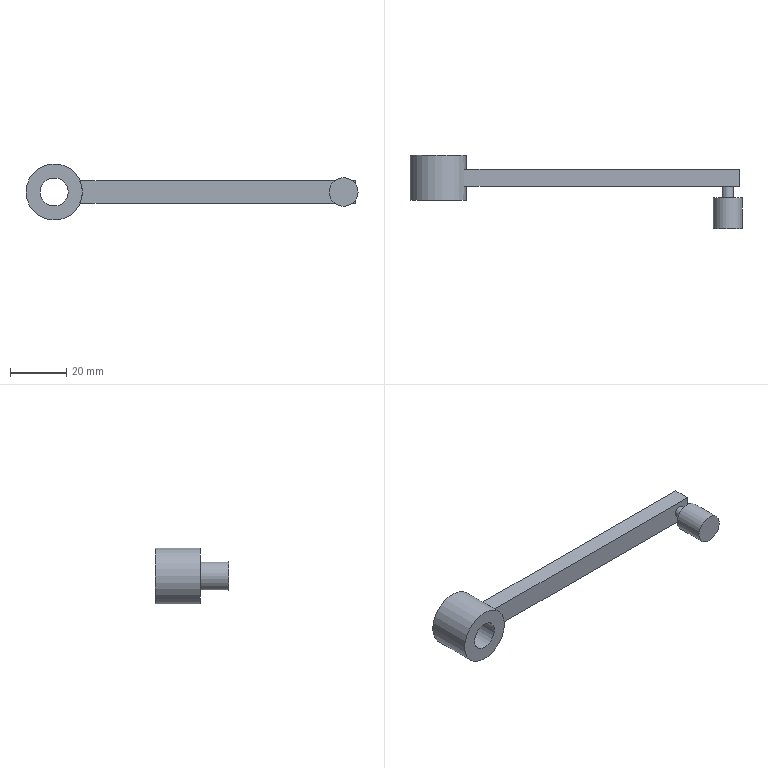Component | NX | HANDRAIL | 1 solid | 13 faces | box 117.89 x 26 x 20 mm | volume 9384 mm3 | plane 9 | cylinder 4 | commonest cylinder face diameters 20 x1 10 x1 4 x1 10.179 x1
STEP:
#1=CARTESIAN_POINT('',(0.,0.,0.));
#2=DIRECTION('',(0.,0.,1.));
#3=DIRECTION('',(1.,0.,0.));
#4=AXIS2_PLACEMENT_3D('',#1,#2,#3);
#5=CARTESIAN_POINT('',(-86.161,-205.381,46.));
#6=VERTEX_POINT('',#5);
#7=CARTESIAN_POINT('',(-86.161,-199.381,46.));
#8=VERTEX_POINT('',#7);
#9=CARTESIAN_POINT('',(-86.161,-210.381,46.));
#10=DIRECTION('',(0.,1.,0.));
#11=VECTOR('',#10,1.);
#12=LINE('',#9,#11);
#13=CARTESIAN_POINT('',(-95.326,-210.381,50.));
#14=DIRECTION('',(0.,1.,0.));
#15=DIRECTION('',(-1.,0.,0.));
#16=AXIS2_PLACEMENT_3D('',#13,#14,#15);
#17=CYLINDRICAL_SURFACE('',#16,10.);
#18=CARTESIAN_POINT('',(3.553,0.));
#19=DIRECTION('',(0.,1.));
#20=VECTOR('',#19,1.);
#21=LINE('',#18,#20);
#22=(GEOMETRIC_REPRESENTATION_CONTEXT(2)PARAMETRIC_REPRESENTATION_CONTEXT()REPRESENTATION_CONTEXT('',''));
#23=DEFINITIONAL_REPRESENTATION('',(#21),#22);
#24=PCURVE('',#17,#23);
#25=CARTESIAN_POINT('',(-88.326,-205.381,46.));
#26=DIRECTION('',(0.,0.,1.));
#27=DIRECTION('',(0.,-1.,0.));
#28=AXIS2_PLACEMENT_3D('',#25,#26,#27);
#29=PLANE('',#28);
#30=CARTESIAN_POINT('',(5.,2.165));
#31=DIRECTION('',(-1.,0.));
#32=VECTOR('',#31,1.);
#33=LINE('',#30,#32);
#34=(GEOMETRIC_REPRESENTATION_CONTEXT(2)PARAMETRIC_REPRESENTATION_CONTEXT()REPRESENTATION_CONTEXT('',''));
#35=DEFINITIONAL_REPRESENTATION('',(#33),#34);
#36=PCURVE('',#29,#35);
#37=SURFACE_CURVE('',#12,(#24,#36),.PCURVE_S1.);
#38=EDGE_CURVE('',#6,#8,#37,.T.);
#39=ORIENTED_EDGE('',*,*,#38,.F.);
#40=CARTESIAN_POINT('',(-85.326,-205.381,50.));
#41=VERTEX_POINT('',#40);
#42=CARTESIAN_POINT('',(-95.326,-205.381,50.));
#43=DIRECTION('',(0.,-1.,0.));
#44=DIRECTION('',(1.,0.,0.));
#45=AXIS2_PLACEMENT_3D('',#42,#43,#44);
#46=CIRCLE('',#45,10.);
#47=CARTESIAN_POINT('',(9.425,5.));
#48=DIRECTION('',(-1.,0.));
#49=VECTOR('',#48,1.);
#50=LINE('',#47,#49);
#51=(GEOMETRIC_REPRESENTATION_CONTEXT(2)PARAMETRIC_REPRESENTATION_CONTEXT()REPRESENTATION_CONTEXT('',''));
#52=DEFINITIONAL_REPRESENTATION('',(#50),#51);
#53=PCURVE('',#17,#52);
#54=CARTESIAN_POINT('',(-95.326,-205.381,50.));
#55=DIRECTION('',(0.,-1.,0.));
#56=DIRECTION('',(1.,0.,0.));
#57=AXIS2_PLACEMENT_3D('',#54,#55,#56);
#58=PLANE('',#57);
#59=CARTESIAN_POINT('',(0.,0.));
#60=DIRECTION('',(1.,0.));
#61=AXIS2_PLACEMENT_2D('',#59,#60);
#62=CIRCLE('',#61,10.);
#63=(GEOMETRIC_REPRESENTATION_CONTEXT(2)PARAMETRIC_REPRESENTATION_CONTEXT()REPRESENTATION_CONTEXT('',''));
#64=DEFINITIONAL_REPRESENTATION('',(#62),#63);
#65=PCURVE('',#58,#64);
#66=SURFACE_CURVE('',#46,(#53,#65),.PCURVE_S1.);
#67=EDGE_CURVE('',#6,#41,#66,.T.);
#68=ORIENTED_EDGE('',*,*,#67,.T.);
#69=CARTESIAN_POINT('',(-85.326,-210.381,50.));
#70=VERTEX_POINT('',#69);
#71=CARTESIAN_POINT('',(-85.326,-210.381,50.));
#72=CARTESIAN_POINT('',(-85.326,-205.381,50.));
#73=B_SPLINE_CURVE_WITH_KNOTS('',1,(#71,#72),.UNSPECIFIED.,.F.,.F.,(2,2),(0.,5.),.PIECEWISE_BEZIER_KNOTS.);
#74=CARTESIAN_POINT('',(3.142,0.));
#75=DIRECTION('',(0.,1.));
#76=VECTOR('',#75,1.);
#77=LINE('',#74,#76);
#78=(GEOMETRIC_REPRESENTATION_CONTEXT(2)PARAMETRIC_REPRESENTATION_CONTEXT()REPRESENTATION_CONTEXT('',''));
#79=DEFINITIONAL_REPRESENTATION('',(#77),#78);
#80=PCURVE('',#17,#79);
#81=CARTESIAN_POINT('',(9.425,0.));
#82=DIRECTION('',(0.,1.));
#83=VECTOR('',#82,1.);
#84=LINE('',#81,#83);
#85=(GEOMETRIC_REPRESENTATION_CONTEXT(2)PARAMETRIC_REPRESENTATION_CONTEXT()REPRESENTATION_CONTEXT('',''));
#86=DEFINITIONAL_REPRESENTATION('',(#84),#85);
#87=PCURVE('',#17,#86);
#88=SEAM_CURVE('',#73,(#80,#87),.PCURVE_S1.);
#89=EDGE_CURVE('',#70,#41,#88,.T.);
#90=ORIENTED_EDGE('',*,*,#89,.F.);
#91=CARTESIAN_POINT('',(-95.326,-210.381,50.));
#92=DIRECTION('',(0.,-1.,0.));
#93=DIRECTION('',(1.,0.,0.));
#94=AXIS2_PLACEMENT_3D('',#91,#92,#93);
#95=CIRCLE('',#94,10.);
#96=CARTESIAN_POINT('',(9.425,0.));
#97=DIRECTION('',(-1.,0.));
#98=VECTOR('',#97,1.);
#99=LINE('',#96,#98);
#100=(GEOMETRIC_REPRESENTATION_CONTEXT(2)PARAMETRIC_REPRESENTATION_CONTEXT()REPRESENTATION_CONTEXT('',''));
#101=DEFINITIONAL_REPRESENTATION('',(#99),#100);
#102=PCURVE('',#17,#101);
#103=CARTESIAN_POINT('',(-95.326,-210.381,50.));
#104=DIRECTION('',(0.,-1.,0.));
#105=DIRECTION('',(1.,0.,0.));
#106=AXIS2_PLACEMENT_3D('',#103,#104,#105);
#107=PLANE('',#106);
#108=CARTESIAN_POINT('',(0.,0.));
#109=DIRECTION('',(1.,0.));
#110=AXIS2_PLACEMENT_2D('',#108,#109);
#111=CIRCLE('',#110,10.);
#112=(GEOMETRIC_REPRESENTATION_CONTEXT(2)PARAMETRIC_REPRESENTATION_CONTEXT()REPRESENTATION_CONTEXT('',''));
#113=DEFINITIONAL_REPRESENTATION('',(#111),#112);
#114=PCURVE('',#107,#113);
#115=SURFACE_CURVE('',#95,(#102,#114),.PCURVE_S1.);
#116=EDGE_CURVE('',#70,#70,#115,.T.);
#117=ORIENTED_EDGE('',*,*,#116,.F.);
#118=ORIENTED_EDGE('',*,*,#89,.T.);
#119=CARTESIAN_POINT('',(-86.161,-205.381,54.));
#120=VERTEX_POINT('',#119);
#121=CARTESIAN_POINT('',(-95.326,-205.381,50.));
#122=DIRECTION('',(0.,-1.,0.));
#123=DIRECTION('',(1.,0.,0.));
#124=AXIS2_PLACEMENT_3D('',#121,#122,#123);
#125=CIRCLE('',#124,10.);
#126=CARTESIAN_POINT('',(15.708,5.));
#127=DIRECTION('',(-1.,0.));
#128=VECTOR('',#127,1.);
#129=LINE('',#126,#128);
#130=(GEOMETRIC_REPRESENTATION_CONTEXT(2)PARAMETRIC_REPRESENTATION_CONTEXT()REPRESENTATION_CONTEXT('',''));
#131=DEFINITIONAL_REPRESENTATION('',(#129),#130);
#132=PCURVE('',#17,#131);
#133=CARTESIAN_POINT('',(0.,0.));
#134=DIRECTION('',(1.,0.));
#135=AXIS2_PLACEMENT_2D('',#133,#134);
#136=CIRCLE('',#135,10.);
#137=(GEOMETRIC_REPRESENTATION_CONTEXT(2)PARAMETRIC_REPRESENTATION_CONTEXT()REPRESENTATION_CONTEXT('',''));
#138=DEFINITIONAL_REPRESENTATION('',(#136),#137);
#139=PCURVE('',#58,#138);
#140=SURFACE_CURVE('',#125,(#132,#139),.PCURVE_S1.);
#141=EDGE_CURVE('',#41,#120,#140,.T.);
#142=ORIENTED_EDGE('',*,*,#141,.T.);
#143=CARTESIAN_POINT('',(-86.161,-199.381,54.));
#144=VERTEX_POINT('',#143);
#145=CARTESIAN_POINT('',(-86.161,-210.381,54.));
#146=DIRECTION('',(0.,-1.,0.));
#147=VECTOR('',#146,1.);
#148=LINE('',#145,#147);
#149=CARTESIAN_POINT('',(9.013,0.));
#150=DIRECTION('',(0.,-1.));
#151=VECTOR('',#150,1.);
#152=LINE('',#149,#151);
#153=(GEOMETRIC_REPRESENTATION_CONTEXT(2)PARAMETRIC_REPRESENTATION_CONTEXT()REPRESENTATION_CONTEXT('',''));
#154=DEFINITIONAL_REPRESENTATION('',(#152),#153);
#155=PCURVE('',#17,#154);
#156=CARTESIAN_POINT('',(11.674,-205.381,54.));
#157=DIRECTION('',(0.,0.,-1.));
#158=DIRECTION('',(0.,1.,0.));
#159=AXIS2_PLACEMENT_3D('',#156,#157,#158);
#160=PLANE('',#159);
#161=CARTESIAN_POINT('',(-5.,-97.835));
#162=DIRECTION('',(-1.,0.));
#163=VECTOR('',#162,1.);
#164=LINE('',#161,#163);
#165=(GEOMETRIC_REPRESENTATION_CONTEXT(2)PARAMETRIC_REPRESENTATION_CONTEXT()REPRESENTATION_CONTEXT('',''));
#166=DEFINITIONAL_REPRESENTATION('',(#164),#165);
#167=PCURVE('',#160,#166);
#168=SURFACE_CURVE('',#148,(#155,#167),.PCURVE_S1.);
#169=EDGE_CURVE('',#144,#120,#168,.T.);
#170=ORIENTED_EDGE('',*,*,#169,.F.);
#171=CARTESIAN_POINT('',(-85.326,-199.381,50.));
#172=VERTEX_POINT('',#171);
#173=CARTESIAN_POINT('',(-95.326,-199.381,50.));
#174=DIRECTION('',(0.,-1.,0.));
#175=DIRECTION('',(1.,0.,0.));
#176=AXIS2_PLACEMENT_3D('',#173,#174,#175);
#177=CIRCLE('',#176,10.);
#178=CARTESIAN_POINT('',(15.708,11.));
#179=DIRECTION('',(-1.,0.));
#180=VECTOR('',#179,1.);
#181=LINE('',#178,#180);
#182=(GEOMETRIC_REPRESENTATION_CONTEXT(2)PARAMETRIC_REPRESENTATION_CONTEXT()REPRESENTATION_CONTEXT('',''));
#183=DEFINITIONAL_REPRESENTATION('',(#181),#182);
#184=PCURVE('',#17,#183);
#185=CARTESIAN_POINT('',(-95.326,-199.381,50.));
#186=DIRECTION('',(0.,-1.,0.));
#187=DIRECTION('',(1.,0.,0.));
#188=AXIS2_PLACEMENT_3D('',#185,#186,#187);
#189=PLANE('',#188);
#190=CARTESIAN_POINT('',(0.,0.));
#191=DIRECTION('',(1.,0.));
#192=AXIS2_PLACEMENT_2D('',#190,#191);
#193=CIRCLE('',#192,10.);
#194=(GEOMETRIC_REPRESENTATION_CONTEXT(2)PARAMETRIC_REPRESENTATION_CONTEXT()REPRESENTATION_CONTEXT('',''));
#195=DEFINITIONAL_REPRESENTATION('',(#193),#194);
#196=PCURVE('',#189,#195);
#197=SURFACE_CURVE('',#177,(#184,#196),.PCURVE_S1.);
#198=EDGE_CURVE('',#172,#144,#197,.T.);
#199=ORIENTED_EDGE('',*,*,#198,.F.);
#200=CARTESIAN_POINT('',(-85.326,-194.381,50.));
#201=VERTEX_POINT('',#200);
#202=CARTESIAN_POINT('',(-85.326,-199.381,50.));
#203=CARTESIAN_POINT('',(-85.326,-194.381,50.));
#204=B_SPLINE_CURVE_WITH_KNOTS('',1,(#202,#203),.UNSPECIFIED.,.F.,.F.,(2,2),(11.,16.),.PIECEWISE_BEZIER_KNOTS.);
#205=CARTESIAN_POINT('',(9.425,0.));
#206=DIRECTION('',(0.,1.));
#207=VECTOR('',#206,1.);
#208=LINE('',#205,#207);
#209=(GEOMETRIC_REPRESENTATION_CONTEXT(2)PARAMETRIC_REPRESENTATION_CONTEXT()REPRESENTATION_CONTEXT('',''));
#210=DEFINITIONAL_REPRESENTATION('',(#208),#209);
#211=PCURVE('',#17,#210);
#212=CARTESIAN_POINT('',(3.142,0.));
#213=DIRECTION('',(0.,1.));
#214=VECTOR('',#213,1.);
#215=LINE('',#212,#214);
#216=(GEOMETRIC_REPRESENTATION_CONTEXT(2)PARAMETRIC_REPRESENTATION_CONTEXT()REPRESENTATION_CONTEXT('',''));
#217=DEFINITIONAL_REPRESENTATION('',(#215),#216);
#218=PCURVE('',#17,#217);
#219=SEAM_CURVE('',#204,(#211,#218),.PCURVE_S1.);
#220=EDGE_CURVE('',#172,#201,#219,.T.);
#221=ORIENTED_EDGE('',*,*,#220,.T.);
#222=CARTESIAN_POINT('',(-95.326,-194.381,50.));
#223=DIRECTION('',(0.,-1.,0.));
#224=DIRECTION('',(1.,0.,0.));
#225=AXIS2_PLACEMENT_3D('',#222,#223,#224);
#226=CIRCLE('',#225,10.);
#227=CARTESIAN_POINT('',(9.425,16.));
#228=DIRECTION('',(-1.,0.));
#229=VECTOR('',#228,1.);
#230=LINE('',#227,#229);
#231=(GEOMETRIC_REPRESENTATION_CONTEXT(2)PARAMETRIC_REPRESENTATION_CONTEXT()REPRESENTATION_CONTEXT('',''));
#232=DEFINITIONAL_REPRESENTATION('',(#230),#231);
#233=PCURVE('',#17,#232);
#234=CARTESIAN_POINT('',(-95.326,-194.381,50.));
#235=DIRECTION('',(0.,-1.,0.));
#236=DIRECTION('',(1.,0.,0.));
#237=AXIS2_PLACEMENT_3D('',#234,#235,#236);
#238=PLANE('',#237);
#239=CARTESIAN_POINT('',(0.,0.));
#240=DIRECTION('',(1.,0.));
#241=AXIS2_PLACEMENT_2D('',#239,#240);
#242=CIRCLE('',#241,10.);
#243=(GEOMETRIC_REPRESENTATION_CONTEXT(2)PARAMETRIC_REPRESENTATION_CONTEXT()REPRESENTATION_CONTEXT('',''));
#244=DEFINITIONAL_REPRESENTATION('',(#242),#243);
#245=PCURVE('',#238,#244);
#246=SURFACE_CURVE('',#226,(#233,#245),.PCURVE_S1.);
#247=EDGE_CURVE('',#201,#201,#246,.T.);
#248=ORIENTED_EDGE('',*,*,#247,.T.);
#249=ORIENTED_EDGE('',*,*,#220,.F.);
#250=CARTESIAN_POINT('',(-95.326,-199.381,50.));
#251=DIRECTION('',(0.,-1.,0.));
#252=DIRECTION('',(1.,0.,0.));
#253=AXIS2_PLACEMENT_3D('',#250,#251,#252);
#254=CIRCLE('',#253,10.);
#255=CARTESIAN_POINT('',(9.425,11.));
#256=DIRECTION('',(-1.,0.));
#257=VECTOR('',#256,1.);
#258=LINE('',#255,#257);
#259=(GEOMETRIC_REPRESENTATION_CONTEXT(2)PARAMETRIC_REPRESENTATION_CONTEXT()REPRESENTATION_CONTEXT('',''));
#260=DEFINITIONAL_REPRESENTATION('',(#258),#259);
#261=PCURVE('',#17,#260);
#262=CARTESIAN_POINT('',(0.,0.));
#263=DIRECTION('',(1.,0.));
#264=AXIS2_PLACEMENT_2D('',#262,#263);
#265=CIRCLE('',#264,10.);
#266=(GEOMETRIC_REPRESENTATION_CONTEXT(2)PARAMETRIC_REPRESENTATION_CONTEXT()REPRESENTATION_CONTEXT('',''));
#267=DEFINITIONAL_REPRESENTATION('',(#265),#266);
#268=PCURVE('',#189,#267);
#269=SURFACE_CURVE('',#254,(#261,#268),.PCURVE_S1.);
#270=EDGE_CURVE('',#8,#172,#269,.T.);
#271=ORIENTED_EDGE('',*,*,#270,.F.);
#272=EDGE_LOOP('',(#39,#68,#90,#117,#118,#142,#170,#199,#221,#248,#249,#271));
#273=FACE_BOUND('',#272,.T.);
#274=ADVANCED_FACE('',(#273),#17,.T.);
#275=CARTESIAN_POINT('',(-90.326,-210.381,50.));
#276=VERTEX_POINT('',#275);
#277=CARTESIAN_POINT('',(-95.326,-210.381,50.));
#278=DIRECTION('',(0.,-1.,0.));
#279=DIRECTION('',(1.,0.,0.));
#280=AXIS2_PLACEMENT_3D('',#277,#278,#279);
#281=CIRCLE('',#280,5.);
#282=CARTESIAN_POINT('',(-95.326,-210.381,50.));
#283=DIRECTION('',(0.,1.,0.));
#284=DIRECTION('',(-1.,0.,0.));
#285=AXIS2_PLACEMENT_3D('',#282,#283,#284);
#286=CYLINDRICAL_SURFACE('',#285,5.);
#287=CARTESIAN_POINT('',(9.425,0.));
#288=DIRECTION('',(-1.,0.));
#289=VECTOR('',#288,1.);
#290=LINE('',#287,#289);
#291=(GEOMETRIC_REPRESENTATION_CONTEXT(2)PARAMETRIC_REPRESENTATION_CONTEXT()REPRESENTATION_CONTEXT('',''));
#292=DEFINITIONAL_REPRESENTATION('',(#290),#291);
#293=PCURVE('',#286,#292);
#294=CARTESIAN_POINT('',(0.,0.));
#295=DIRECTION('',(1.,0.));
#296=AXIS2_PLACEMENT_2D('',#294,#295);
#297=CIRCLE('',#296,5.);
#298=(GEOMETRIC_REPRESENTATION_CONTEXT(2)PARAMETRIC_REPRESENTATION_CONTEXT()REPRESENTATION_CONTEXT('',''));
#299=DEFINITIONAL_REPRESENTATION('',(#297),#298);
#300=PCURVE('',#107,#299);
#301=SURFACE_CURVE('',#281,(#293,#300),.PCURVE_S1.);
#302=EDGE_CURVE('',#276,#276,#301,.T.);
#303=ORIENTED_EDGE('',*,*,#302,.F.);
#304=CARTESIAN_POINT('',(-90.326,-194.381,50.));
#305=VERTEX_POINT('',#304);
#306=CARTESIAN_POINT('',(-90.326,-210.381,50.));
#307=CARTESIAN_POINT('',(-90.326,-194.381,50.));
#308=B_SPLINE_CURVE_WITH_KNOTS('',1,(#306,#307),.UNSPECIFIED.,.F.,.F.,(2,2),(0.,16.),.PIECEWISE_BEZIER_KNOTS.);
#309=CARTESIAN_POINT('',(9.425,0.));
#310=DIRECTION('',(0.,1.));
#311=VECTOR('',#310,1.);
#312=LINE('',#309,#311);
#313=(GEOMETRIC_REPRESENTATION_CONTEXT(2)PARAMETRIC_REPRESENTATION_CONTEXT()REPRESENTATION_CONTEXT('',''));
#314=DEFINITIONAL_REPRESENTATION('',(#312),#313);
#315=PCURVE('',#286,#314);
#316=CARTESIAN_POINT('',(3.142,0.));
#317=DIRECTION('',(0.,1.));
#318=VECTOR('',#317,1.);
#319=LINE('',#316,#318);
#320=(GEOMETRIC_REPRESENTATION_CONTEXT(2)PARAMETRIC_REPRESENTATION_CONTEXT()REPRESENTATION_CONTEXT('',''));
#321=DEFINITIONAL_REPRESENTATION('',(#319),#320);
#322=PCURVE('',#286,#321);
#323=SEAM_CURVE('',#308,(#315,#322),.PCURVE_S1.);
#324=EDGE_CURVE('',#276,#305,#323,.T.);
#325=ORIENTED_EDGE('',*,*,#324,.T.);
#326=CARTESIAN_POINT('',(-95.326,-194.381,50.));
#327=DIRECTION('',(0.,-1.,0.));
#328=DIRECTION('',(1.,0.,0.));
#329=AXIS2_PLACEMENT_3D('',#326,#327,#328);
#330=CIRCLE('',#329,5.);
#331=CARTESIAN_POINT('',(9.425,16.));
#332=DIRECTION('',(-1.,0.));
#333=VECTOR('',#332,1.);
#334=LINE('',#331,#333);
#335=(GEOMETRIC_REPRESENTATION_CONTEXT(2)PARAMETRIC_REPRESENTATION_CONTEXT()REPRESENTATION_CONTEXT('',''));
#336=DEFINITIONAL_REPRESENTATION('',(#334),#335);
#337=PCURVE('',#286,#336);
#338=CARTESIAN_POINT('',(0.,0.));
#339=DIRECTION('',(1.,0.));
#340=AXIS2_PLACEMENT_2D('',#338,#339);
#341=CIRCLE('',#340,5.);
#342=(GEOMETRIC_REPRESENTATION_CONTEXT(2)PARAMETRIC_REPRESENTATION_CONTEXT()REPRESENTATION_CONTEXT('',''));
#343=DEFINITIONAL_REPRESENTATION('',(#341),#342);
#344=PCURVE('',#238,#343);
#345=SURFACE_CURVE('',#330,(#337,#344),.PCURVE_S1.);
#346=EDGE_CURVE('',#305,#305,#345,.T.);
#347=ORIENTED_EDGE('',*,*,#346,.T.);
#348=ORIENTED_EDGE('',*,*,#324,.F.);
#349=EDGE_LOOP('',(#303,#325,#347,#348));
#350=FACE_BOUND('',#349,.F.);
#351=ADVANCED_FACE('',(#350),#286,.F.);
#352=ORIENTED_EDGE('',*,*,#116,.T.);
#353=EDGE_LOOP('',(#352));
#354=FACE_BOUND('',#353,.T.);
#355=ORIENTED_EDGE('',*,*,#302,.F.);
#356=EDGE_LOOP('',(#355));
#357=FACE_BOUND('',#356,.T.);
#358=ADVANCED_FACE('',(#354,#357),#107,.T.);
#359=ORIENTED_EDGE('',*,*,#247,.F.);
#360=EDGE_LOOP('',(#359));
#361=FACE_BOUND('',#360,.T.);
#362=ORIENTED_EDGE('',*,*,#346,.T.);
#363=EDGE_LOOP('',(#362));
#364=FACE_BOUND('',#363,.T.);
#365=ADVANCED_FACE('',(#361,#364),#238,.F.);
#366=CARTESIAN_POINT('',(11.674,-205.381,46.));
#367=VERTEX_POINT('',#366);
#368=CARTESIAN_POINT('',(-88.326,-205.381,46.));
#369=DIRECTION('',(1.,0.,0.));
#370=VECTOR('',#369,1.);
#371=LINE('',#368,#370);
#372=CARTESIAN_POINT('',(0.,0.));
#373=DIRECTION('',(0.,1.));
#374=VECTOR('',#373,1.);
#375=LINE('',#372,#374);
#376=(GEOMETRIC_REPRESENTATION_CONTEXT(2)PARAMETRIC_REPRESENTATION_CONTEXT()REPRESENTATION_CONTEXT('',''));
#377=DEFINITIONAL_REPRESENTATION('',(#375),#376);
#378=PCURVE('',#29,#377);
#379=CARTESIAN_POINT('',(7.,-4.));
#380=DIRECTION('',(1.,0.));
#381=VECTOR('',#380,1.);
#382=LINE('',#379,#381);
#383=(GEOMETRIC_REPRESENTATION_CONTEXT(2)PARAMETRIC_REPRESENTATION_CONTEXT()REPRESENTATION_CONTEXT('',''));
#384=DEFINITIONAL_REPRESENTATION('',(#382),#383);
#385=PCURVE('',#58,#384);
#386=SURFACE_CURVE('',#371,(#378,#385),.PCURVE_S1.);
#387=EDGE_CURVE('',#6,#367,#386,.T.);
#388=ORIENTED_EDGE('',*,*,#387,.F.);
#389=ORIENTED_EDGE('',*,*,#38,.T.);
#390=CARTESIAN_POINT('',(11.674,-199.381,46.));
#391=VERTEX_POINT('',#390);
#392=CARTESIAN_POINT('',(-88.326,-199.381,46.));
#393=DIRECTION('',(1.,0.,0.));
#394=VECTOR('',#393,1.);
#395=LINE('',#392,#394);
#396=CARTESIAN_POINT('',(-6.,0.));
#397=DIRECTION('',(0.,1.));
#398=VECTOR('',#397,1.);
#399=LINE('',#396,#398);
#400=(GEOMETRIC_REPRESENTATION_CONTEXT(2)PARAMETRIC_REPRESENTATION_CONTEXT()REPRESENTATION_CONTEXT('',''));
#401=DEFINITIONAL_REPRESENTATION('',(#399),#400);
#402=PCURVE('',#29,#401);
#403=CARTESIAN_POINT('',(7.,-4.));
#404=DIRECTION('',(1.,0.));
#405=VECTOR('',#404,1.);
#406=LINE('',#403,#405);
#407=(GEOMETRIC_REPRESENTATION_CONTEXT(2)PARAMETRIC_REPRESENTATION_CONTEXT()REPRESENTATION_CONTEXT('',''));
#408=DEFINITIONAL_REPRESENTATION('',(#406),#407);
#409=PCURVE('',#189,#408);
#410=SURFACE_CURVE('',#395,(#402,#409),.PCURVE_S1.);
#411=EDGE_CURVE('',#8,#391,#410,.T.);
#412=ORIENTED_EDGE('',*,*,#411,.T.);
#413=CARTESIAN_POINT('',(11.674,-205.381,46.));
#414=DIRECTION('',(0.,1.,0.));
#415=VECTOR('',#414,1.);
#416=LINE('',#413,#415);
#417=CARTESIAN_POINT('',(0.,100.));
#418=DIRECTION('',(-1.,0.));
#419=VECTOR('',#418,1.);
#420=LINE('',#417,#419);
#421=(GEOMETRIC_REPRESENTATION_CONTEXT(2)PARAMETRIC_REPRESENTATION_CONTEXT()REPRESENTATION_CONTEXT('',''));
#422=DEFINITIONAL_REPRESENTATION('',(#420),#421);
#423=PCURVE('',#29,#422);
#424=CARTESIAN_POINT('',(11.674,-205.381,50.));
#425=DIRECTION('',(-1.,0.,0.));
#426=DIRECTION('',(0.,-1.,0.));
#427=AXIS2_PLACEMENT_3D('',#424,#425,#426);
#428=PLANE('',#427);
#429=CARTESIAN_POINT('',(0.,-4.));
#430=DIRECTION('',(-1.,0.));
#431=VECTOR('',#430,1.);
#432=LINE('',#429,#431);
#433=(GEOMETRIC_REPRESENTATION_CONTEXT(2)PARAMETRIC_REPRESENTATION_CONTEXT()REPRESENTATION_CONTEXT('',''));
#434=DEFINITIONAL_REPRESENTATION('',(#432),#433);
#435=PCURVE('',#428,#434);
#436=SURFACE_CURVE('',#416,(#423,#435),.PCURVE_S1.);
#437=EDGE_CURVE('',#367,#391,#436,.T.);
#438=ORIENTED_EDGE('',*,*,#437,.F.);
#439=EDGE_LOOP('',(#388,#389,#412,#438));
#440=FACE_BOUND('',#439,.T.);
#441=ADVANCED_FACE('',(#440),#29,.F.);
#442=CARTESIAN_POINT('',(11.674,-199.381,54.));
#443=VERTEX_POINT('',#442);
#444=CARTESIAN_POINT('',(11.674,-199.381,54.));
#445=DIRECTION('',(-1.,0.,0.));
#446=VECTOR('',#445,1.);
#447=LINE('',#444,#446);
#448=CARTESIAN_POINT('',(6.,0.));
#449=DIRECTION('',(0.,-1.));
#450=VECTOR('',#449,1.);
#451=LINE('',#448,#450);
#452=(GEOMETRIC_REPRESENTATION_CONTEXT(2)PARAMETRIC_REPRESENTATION_CONTEXT()REPRESENTATION_CONTEXT('',''));
#453=DEFINITIONAL_REPRESENTATION('',(#451),#452);
#454=PCURVE('',#160,#453);
#455=CARTESIAN_POINT('',(107.,4.));
#456=DIRECTION('',(-1.,0.));
#457=VECTOR('',#456,1.);
#458=LINE('',#455,#457);
#459=(GEOMETRIC_REPRESENTATION_CONTEXT(2)PARAMETRIC_REPRESENTATION_CONTEXT()REPRESENTATION_CONTEXT('',''));
#460=DEFINITIONAL_REPRESENTATION('',(#458),#459);
#461=PCURVE('',#189,#460);
#462=SURFACE_CURVE('',#447,(#454,#461),.PCURVE_S1.);
#463=EDGE_CURVE('',#443,#144,#462,.T.);
#464=ORIENTED_EDGE('',*,*,#463,.T.);
#465=ORIENTED_EDGE('',*,*,#169,.T.);
#466=CARTESIAN_POINT('',(11.674,-205.381,54.));
#467=VERTEX_POINT('',#466);
#468=CARTESIAN_POINT('',(11.674,-205.381,54.));
#469=DIRECTION('',(-1.,0.,0.));
#470=VECTOR('',#469,1.);
#471=LINE('',#468,#470);
#472=CARTESIAN_POINT('',(0.,0.));
#473=DIRECTION('',(0.,-1.));
#474=VECTOR('',#473,1.);
#475=LINE('',#472,#474);
#476=(GEOMETRIC_REPRESENTATION_CONTEXT(2)PARAMETRIC_REPRESENTATION_CONTEXT()REPRESENTATION_CONTEXT('',''));
#477=DEFINITIONAL_REPRESENTATION('',(#475),#476);
#478=PCURVE('',#160,#477);
#479=CARTESIAN_POINT('',(107.,4.));
#480=DIRECTION('',(-1.,0.));
#481=VECTOR('',#480,1.);
#482=LINE('',#479,#481);
#483=(GEOMETRIC_REPRESENTATION_CONTEXT(2)PARAMETRIC_REPRESENTATION_CONTEXT()REPRESENTATION_CONTEXT('',''));
#484=DEFINITIONAL_REPRESENTATION('',(#482),#483);
#485=PCURVE('',#58,#484);
#486=SURFACE_CURVE('',#471,(#478,#485),.PCURVE_S1.);
#487=EDGE_CURVE('',#467,#120,#486,.T.);
#488=ORIENTED_EDGE('',*,*,#487,.F.);
#489=CARTESIAN_POINT('',(11.674,-205.381,54.));
#490=DIRECTION('',(0.,1.,0.));
#491=VECTOR('',#490,1.);
#492=LINE('',#489,#491);
#493=CARTESIAN_POINT('',(0.,0.));
#494=DIRECTION('',(1.,0.));
#495=VECTOR('',#494,1.);
#496=LINE('',#493,#495);
#497=(GEOMETRIC_REPRESENTATION_CONTEXT(2)PARAMETRIC_REPRESENTATION_CONTEXT()REPRESENTATION_CONTEXT('',''));
#498=DEFINITIONAL_REPRESENTATION('',(#496),#497);
#499=PCURVE('',#160,#498);
#500=CARTESIAN_POINT('',(0.,4.));
#501=DIRECTION('',(-1.,0.));
#502=VECTOR('',#501,1.);
#503=LINE('',#500,#502);
#504=(GEOMETRIC_REPRESENTATION_CONTEXT(2)PARAMETRIC_REPRESENTATION_CONTEXT()REPRESENTATION_CONTEXT('',''));
#505=DEFINITIONAL_REPRESENTATION('',(#503),#504);
#506=PCURVE('',#428,#505);
#507=SURFACE_CURVE('',#492,(#499,#506),.PCURVE_S1.);
#508=EDGE_CURVE('',#467,#443,#507,.T.);
#509=ORIENTED_EDGE('',*,*,#508,.T.);
#510=EDGE_LOOP('',(#464,#465,#488,#509));
#511=FACE_BOUND('',#510,.T.);
#512=ADVANCED_FACE('',(#511),#160,.F.);
#513=CARTESIAN_POINT('',(11.674,-199.381,50.));
#514=DIRECTION('',(0.,0.,1.));
#515=VECTOR('',#514,1.);
#516=LINE('',#513,#515);
#517=CARTESIAN_POINT('',(-6.,0.));
#518=DIRECTION('',(0.,1.));
#519=VECTOR('',#518,1.);
#520=LINE('',#517,#519);
#521=(GEOMETRIC_REPRESENTATION_CONTEXT(2)PARAMETRIC_REPRESENTATION_CONTEXT()REPRESENTATION_CONTEXT('',''));
#522=DEFINITIONAL_REPRESENTATION('',(#520),#521);
#523=PCURVE('',#428,#522);
#524=CARTESIAN_POINT('',(107.,0.));
#525=DIRECTION('',(0.,1.));
#526=VECTOR('',#525,1.);
#527=LINE('',#524,#526);
#528=(GEOMETRIC_REPRESENTATION_CONTEXT(2)PARAMETRIC_REPRESENTATION_CONTEXT()REPRESENTATION_CONTEXT('',''));
#529=DEFINITIONAL_REPRESENTATION('',(#527),#528);
#530=PCURVE('',#189,#529);
#531=SURFACE_CURVE('',#516,(#523,#530),.PCURVE_S1.);
#532=EDGE_CURVE('',#391,#443,#531,.T.);
#533=ORIENTED_EDGE('',*,*,#532,.T.);
#534=ORIENTED_EDGE('',*,*,#508,.F.);
#535=CARTESIAN_POINT('',(11.674,-205.381,46.));
#536=DIRECTION('',(0.,0.,1.));
#537=VECTOR('',#536,1.);
#538=LINE('',#535,#537);
#539=CARTESIAN_POINT('',(0.,-4.));
#540=DIRECTION('',(0.,1.));
#541=VECTOR('',#540,1.);
#542=LINE('',#539,#541);
#543=(GEOMETRIC_REPRESENTATION_CONTEXT(2)PARAMETRIC_REPRESENTATION_CONTEXT()REPRESENTATION_CONTEXT('',''));
#544=DEFINITIONAL_REPRESENTATION('',(#542),#543);
#545=PCURVE('',#428,#544);
#546=CARTESIAN_POINT('',(107.,-4.));
#547=DIRECTION('',(0.,1.));
#548=VECTOR('',#547,1.);
#549=LINE('',#546,#548);
#550=(GEOMETRIC_REPRESENTATION_CONTEXT(2)PARAMETRIC_REPRESENTATION_CONTEXT()REPRESENTATION_CONTEXT('',''));
#551=DEFINITIONAL_REPRESENTATION('',(#549),#550);
#552=PCURVE('',#58,#551);
#553=SURFACE_CURVE('',#538,(#545,#552),.PCURVE_S1.);
#554=EDGE_CURVE('',#367,#467,#553,.T.);
#555=ORIENTED_EDGE('',*,*,#554,.F.);
#556=ORIENTED_EDGE('',*,*,#437,.T.);
#557=EDGE_LOOP('',(#533,#534,#555,#556));
#558=FACE_BOUND('',#557,.T.);
#559=ADVANCED_FACE('',(#558),#428,.F.);
#560=CARTESIAN_POINT('',(9.477,-205.381,50.));
#561=VERTEX_POINT('',#560);
#562=CARTESIAN_POINT('',(7.477,-205.381,50.));
#563=DIRECTION('',(0.,-1.,0.));
#564=DIRECTION('',(1.,0.,0.));
#565=AXIS2_PLACEMENT_3D('',#562,#563,#564);
#566=CIRCLE('',#565,2.);
#567=CARTESIAN_POINT('',(102.803,0.));
#568=DIRECTION('',(1.,0.));
#569=AXIS2_PLACEMENT_2D('',#567,#568);
#570=CIRCLE('',#569,2.);
#571=(GEOMETRIC_REPRESENTATION_CONTEXT(2)PARAMETRIC_REPRESENTATION_CONTEXT()REPRESENTATION_CONTEXT('',''));
#572=DEFINITIONAL_REPRESENTATION('',(#570),#571);
#573=PCURVE('',#58,#572);
#574=CARTESIAN_POINT('',(7.477,-209.381,50.));
#575=DIRECTION('',(0.,1.,0.));
#576=DIRECTION('',(-1.,0.,0.));
#577=AXIS2_PLACEMENT_3D('',#574,#575,#576);
#578=CYLINDRICAL_SURFACE('',#577,2.);
#579=CARTESIAN_POINT('',(9.425,4.));
#580=DIRECTION('',(-1.,0.));
#581=VECTOR('',#580,1.);
#582=LINE('',#579,#581);
#583=(GEOMETRIC_REPRESENTATION_CONTEXT(2)PARAMETRIC_REPRESENTATION_CONTEXT()REPRESENTATION_CONTEXT('',''));
#584=DEFINITIONAL_REPRESENTATION('',(#582),#583);
#585=PCURVE('',#578,#584);
#586=SURFACE_CURVE('',#566,(#573,#585),.PCURVE_S1.);
#587=EDGE_CURVE('',#561,#561,#586,.T.);
#588=ORIENTED_EDGE('',*,*,#587,.F.);
#589=EDGE_LOOP('',(#588));
#590=FACE_BOUND('',#589,.T.);
#591=ORIENTED_EDGE('',*,*,#67,.F.);
#592=ORIENTED_EDGE('',*,*,#387,.T.);
#593=ORIENTED_EDGE('',*,*,#554,.T.);
#594=ORIENTED_EDGE('',*,*,#487,.T.);
#595=ORIENTED_EDGE('',*,*,#141,.F.);
#596=EDGE_LOOP('',(#591,#592,#593,#594,#595));
#597=FACE_BOUND('',#596,.T.);
#598=ADVANCED_FACE('',(#590,#597),#58,.T.);
#599=ORIENTED_EDGE('',*,*,#411,.F.);
#600=ORIENTED_EDGE('',*,*,#270,.T.);
#601=ORIENTED_EDGE('',*,*,#198,.T.);
#602=ORIENTED_EDGE('',*,*,#463,.F.);
#603=ORIENTED_EDGE('',*,*,#532,.F.);
#604=EDGE_LOOP('',(#599,#600,#601,#602,#603));
#605=FACE_BOUND('',#604,.T.);
#606=ADVANCED_FACE('',(#605),#189,.F.);
#607=CARTESIAN_POINT('',(9.477,-209.381,50.));
#608=VERTEX_POINT('',#607);
#609=CARTESIAN_POINT('',(7.477,-209.381,50.));
#610=DIRECTION('',(0.,-1.,0.));
#611=DIRECTION('',(1.,0.,0.));
#612=AXIS2_PLACEMENT_3D('',#609,#610,#611);
#613=CIRCLE('',#612,2.);
#614=CARTESIAN_POINT('',(9.425,0.));
#615=DIRECTION('',(-1.,0.));
#616=VECTOR('',#615,1.);
#617=LINE('',#614,#616);
#618=(GEOMETRIC_REPRESENTATION_CONTEXT(2)PARAMETRIC_REPRESENTATION_CONTEXT()REPRESENTATION_CONTEXT('',''));
#619=DEFINITIONAL_REPRESENTATION('',(#617),#618);
#620=PCURVE('',#578,#619);
#621=CARTESIAN_POINT('',(7.477,-209.381,50.));
#622=DIRECTION('',(0.,-1.,0.));
#623=DIRECTION('',(1.,0.,0.));
#624=AXIS2_PLACEMENT_3D('',#621,#622,#623);
#625=PLANE('',#624);
#626=CARTESIAN_POINT('',(0.,0.));
#627=DIRECTION('',(1.,0.));
#628=AXIS2_PLACEMENT_2D('',#626,#627);
#629=CIRCLE('',#628,2.);
#630=(GEOMETRIC_REPRESENTATION_CONTEXT(2)PARAMETRIC_REPRESENTATION_CONTEXT()REPRESENTATION_CONTEXT('',''));
#631=DEFINITIONAL_REPRESENTATION('',(#629),#630);
#632=PCURVE('',#625,#631);
#633=SURFACE_CURVE('',#613,(#620,#632),.PCURVE_S1.);
#634=EDGE_CURVE('',#608,#608,#633,.T.);
#635=ORIENTED_EDGE('',*,*,#634,.F.);
#636=CARTESIAN_POINT('',(9.477,-209.381,50.));
#637=CARTESIAN_POINT('',(9.477,-205.381,50.));
#638=B_SPLINE_CURVE_WITH_KNOTS('',1,(#636,#637),.UNSPECIFIED.,.F.,.F.,(2,2),(0.,4.),.PIECEWISE_BEZIER_KNOTS.);
#639=CARTESIAN_POINT('',(9.425,0.));
#640=DIRECTION('',(0.,1.));
#641=VECTOR('',#640,1.);
#642=LINE('',#639,#641);
#643=(GEOMETRIC_REPRESENTATION_CONTEXT(2)PARAMETRIC_REPRESENTATION_CONTEXT()REPRESENTATION_CONTEXT('',''));
#644=DEFINITIONAL_REPRESENTATION('',(#642),#643);
#645=PCURVE('',#578,#644);
#646=CARTESIAN_POINT('',(3.142,0.));
#647=DIRECTION('',(0.,1.));
#648=VECTOR('',#647,1.);
#649=LINE('',#646,#648);
#650=(GEOMETRIC_REPRESENTATION_CONTEXT(2)PARAMETRIC_REPRESENTATION_CONTEXT()REPRESENTATION_CONTEXT('',''));
#651=DEFINITIONAL_REPRESENTATION('',(#649),#650);
#652=PCURVE('',#578,#651);
#653=SEAM_CURVE('',#638,(#645,#652),.PCURVE_S1.);
#654=EDGE_CURVE('',#608,#561,#653,.T.);
#655=ORIENTED_EDGE('',*,*,#654,.T.);
#656=ORIENTED_EDGE('',*,*,#587,.T.);
#657=ORIENTED_EDGE('',*,*,#654,.F.);
#658=EDGE_LOOP('',(#635,#655,#656,#657));
#659=FACE_BOUND('',#658,.T.);
#660=ADVANCED_FACE('',(#659),#578,.T.);
#661=CARTESIAN_POINT('',(12.566,-220.381,50.));
#662=VERTEX_POINT('',#661);
#663=CARTESIAN_POINT('',(7.477,-220.381,50.));
#664=DIRECTION('',(0.,-1.,0.));
#665=DIRECTION('',(1.,0.,0.));
#666=AXIS2_PLACEMENT_3D('',#663,#664,#665);
#667=CIRCLE('',#666,5.09);
#668=CARTESIAN_POINT('',(7.477,-220.381,50.));
#669=DIRECTION('',(0.,1.,0.));
#670=DIRECTION('',(-1.,0.,0.));
#671=AXIS2_PLACEMENT_3D('',#668,#669,#670);
#672=CYLINDRICAL_SURFACE('',#671,5.09);
#673=CARTESIAN_POINT('',(9.425,0.));
#674=DIRECTION('',(-1.,0.));
#675=VECTOR('',#674,1.);
#676=LINE('',#673,#675);
#677=(GEOMETRIC_REPRESENTATION_CONTEXT(2)PARAMETRIC_REPRESENTATION_CONTEXT()REPRESENTATION_CONTEXT('',''));
#678=DEFINITIONAL_REPRESENTATION('',(#676),#677);
#679=PCURVE('',#672,#678);
#680=CARTESIAN_POINT('',(7.477,-220.381,50.));
#681=DIRECTION('',(0.,-1.,0.));
#682=DIRECTION('',(1.,0.,0.));
#683=AXIS2_PLACEMENT_3D('',#680,#681,#682);
#684=PLANE('',#683);
#685=CARTESIAN_POINT('',(0.,0.));
#686=DIRECTION('',(1.,0.));
#687=AXIS2_PLACEMENT_2D('',#685,#686);
#688=CIRCLE('',#687,5.09);
#689=(GEOMETRIC_REPRESENTATION_CONTEXT(2)PARAMETRIC_REPRESENTATION_CONTEXT()REPRESENTATION_CONTEXT('',''));
#690=DEFINITIONAL_REPRESENTATION('',(#688),#689);
#691=PCURVE('',#684,#690);
#692=SURFACE_CURVE('',#667,(#679,#691),.PCURVE_S1.);
#693=EDGE_CURVE('',#662,#662,#692,.T.);
#694=ORIENTED_EDGE('',*,*,#693,.F.);
#695=CARTESIAN_POINT('',(12.566,-209.381,50.));
#696=VERTEX_POINT('',#695);
#697=CARTESIAN_POINT('',(12.566,-220.381,50.));
#698=CARTESIAN_POINT('',(12.566,-209.381,50.));
#699=B_SPLINE_CURVE_WITH_KNOTS('',1,(#697,#698),.UNSPECIFIED.,.F.,.F.,(2,2),(0.,11.),.PIECEWISE_BEZIER_KNOTS.);
#700=CARTESIAN_POINT('',(9.425,0.));
#701=DIRECTION('',(0.,1.));
#702=VECTOR('',#701,1.);
#703=LINE('',#700,#702);
#704=(GEOMETRIC_REPRESENTATION_CONTEXT(2)PARAMETRIC_REPRESENTATION_CONTEXT()REPRESENTATION_CONTEXT('',''));
#705=DEFINITIONAL_REPRESENTATION('',(#703),#704);
#706=PCURVE('',#672,#705);
#707=CARTESIAN_POINT('',(3.142,0.));
#708=DIRECTION('',(0.,1.));
#709=VECTOR('',#708,1.);
#710=LINE('',#707,#709);
#711=(GEOMETRIC_REPRESENTATION_CONTEXT(2)PARAMETRIC_REPRESENTATION_CONTEXT()REPRESENTATION_CONTEXT('',''));
#712=DEFINITIONAL_REPRESENTATION('',(#710),#711);
#713=PCURVE('',#672,#712);
#714=SEAM_CURVE('',#699,(#706,#713),.PCURVE_S1.);
#715=EDGE_CURVE('',#662,#696,#714,.T.);
#716=ORIENTED_EDGE('',*,*,#715,.T.);
#717=CARTESIAN_POINT('',(7.477,-209.381,50.));
#718=DIRECTION('',(0.,-1.,0.));
#719=DIRECTION('',(1.,0.,0.));
#720=AXIS2_PLACEMENT_3D('',#717,#718,#719);
#721=CIRCLE('',#720,5.09);
#722=CARTESIAN_POINT('',(9.425,11.));
#723=DIRECTION('',(-1.,0.));
#724=VECTOR('',#723,1.);
#725=LINE('',#722,#724);
#726=(GEOMETRIC_REPRESENTATION_CONTEXT(2)PARAMETRIC_REPRESENTATION_CONTEXT()REPRESENTATION_CONTEXT('',''));
#727=DEFINITIONAL_REPRESENTATION('',(#725),#726);
#728=PCURVE('',#672,#727);
#729=CARTESIAN_POINT('',(0.,0.));
#730=DIRECTION('',(1.,0.));
#731=AXIS2_PLACEMENT_2D('',#729,#730);
#732=CIRCLE('',#731,5.09);
#733=(GEOMETRIC_REPRESENTATION_CONTEXT(2)PARAMETRIC_REPRESENTATION_CONTEXT()REPRESENTATION_CONTEXT('',''));
#734=DEFINITIONAL_REPRESENTATION('',(#732),#733);
#735=PCURVE('',#625,#734);
#736=SURFACE_CURVE('',#721,(#728,#735),.PCURVE_S1.);
#737=EDGE_CURVE('',#696,#696,#736,.T.);
#738=ORIENTED_EDGE('',*,*,#737,.T.);
#739=ORIENTED_EDGE('',*,*,#715,.F.);
#740=EDGE_LOOP('',(#694,#716,#738,#739));
#741=FACE_BOUND('',#740,.T.);
#742=ADVANCED_FACE('',(#741),#672,.T.);
#743=ORIENTED_EDGE('',*,*,#693,.T.);
#744=EDGE_LOOP('',(#743));
#745=FACE_BOUND('',#744,.T.);
#746=ADVANCED_FACE('',(#745),#684,.T.);
#747=ORIENTED_EDGE('',*,*,#634,.T.);
#748=EDGE_LOOP('',(#747));
#749=FACE_BOUND('',#748,.T.);
#750=ORIENTED_EDGE('',*,*,#737,.F.);
#751=EDGE_LOOP('',(#750));
#752=FACE_BOUND('',#751,.T.);
#753=ADVANCED_FACE('',(#749,#752),#625,.F.);
#754=CLOSED_SHELL('',(#274,#351,#358,#365,#441,#512,#559,#598,#606,#660,#742,#746,#753));
#755=MANIFOLD_SOLID_BREP('',#754);
#756=(LENGTH_UNIT()NAMED_UNIT(*)SI_UNIT(.MILLI.,.METRE.));
#757=UNCERTAINTY_MEASURE_WITH_UNIT(LENGTH_MEASURE(0.000005),#756,'','');
#758=(NAMED_UNIT(*)PLANE_ANGLE_UNIT()SI_UNIT($,.RADIAN.));
#759=(NAMED_UNIT(*)SI_UNIT($,.STERADIAN.)SOLID_ANGLE_UNIT());
#760=(GEOMETRIC_REPRESENTATION_CONTEXT(3)GLOBAL_UNCERTAINTY_ASSIGNED_CONTEXT((#757))GLOBAL_UNIT_ASSIGNED_CONTEXT((#756,#758,#759))REPRESENTATION_CONTEXT('',''));
#761=ADVANCED_BREP_SHAPE_REPRESENTATION('',(#4,#755),#760);